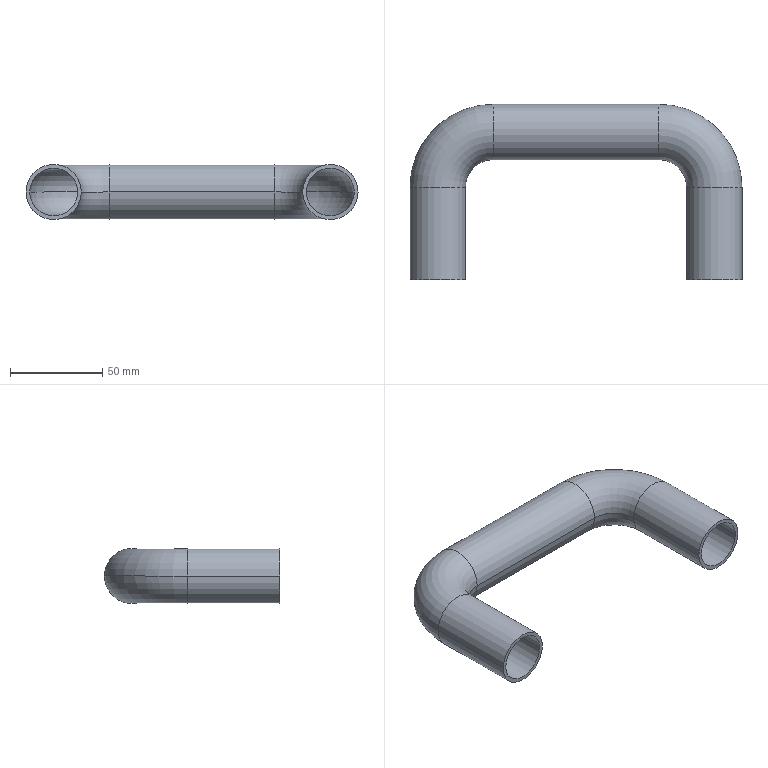Component | SolidWorks | CoverPlate-100_CoverHandle-1 | 1 solid | 22 faces | box 180 x 95 x 30 mm | volume 50007 mm3 | cylinder 12 | torus 8 | plane 2 | commonest cylinder face diameters 26 x6 30 x6 | material Plain Carbon Steel
build123d program:
from build123d import *

# Parameters (mm, degrees)
SWEEP_THIN1_PROFILE_R   = 15
SWEEP_THIN1_PROFILE_R_2 = 13


with BuildPart() as part:
    # Sweep-Thin1: sweep along a path in Sketch1
    with BuildLine(Plane(origin=(0, 0, 0), x_dir=(1, 0, 0), z_dir=(0, 1, 0))) as sweep_thin1_path:
        Line((0, 0), (0, 50))
        ThreePointArc((0, 50), (8.787, 71.213), (30, 80))
        Line((30, 80), (120, 80))
        ThreePointArc((120, 80), (141.213, 71.213), (150, 50))
        Line((150, 50), (150, 0))
    # Sweep-Thin1 profile (on start of the path) → Sweep-Thin1 (sweep)
    with BuildSketch(Plane(origin=(0, 0, 0), x_dir=(-1, 0, 0), z_dir=(0, 0, -1))):
        Circle(SWEEP_THIN1_PROFILE_R)
        Circle(SWEEP_THIN1_PROFILE_R_2, mode=Mode.SUBTRACT)
    sweep(path=sweep_thin1_path.line)


solid = part.part

# Placed as in the assembly
solid = solid.moved(Location((-455.465, 3543.733, 6089.043), (90, 0, 0)))
STEP:
#1=COLOUR_RGB('',0.7922,0.8196,0.9333);
#2=FILL_AREA_STYLE_COLOUR('',#1);
#3=FILL_AREA_STYLE('',(#2));
#4=SURFACE_STYLE_FILL_AREA(#3);
#5=SURFACE_SIDE_STYLE('',(#4));
#6=SURFACE_STYLE_USAGE(.BOTH.,#5);
#7=PRESENTATION_STYLE_ASSIGNMENT((#6));
#8=CARTESIAN_POINT('',(-13.207,142.155,239.726));
#9=VERTEX_POINT('',#8);
#10=CARTESIAN_POINT('',(-13.207,143.178,239.726));
#11=VERTEX_POINT('',#10);
#12=CARTESIAN_POINT('',(-13.207,142.667,239.726));
#13=DIRECTION('',(-1.,0.,0.));
#14=DIRECTION('',(0.,1.,0.));
#15=AXIS2_PLACEMENT_3D('',#12,#13,#14);
#16=CIRCLE('',#15,0.5118);
#17=EDGE_CURVE('',#9,#11,#16,.T.);
#18=ORIENTED_EDGE('',*,*,#17,.T.);
#19=CARTESIAN_POINT('',(-11.514,141.486,239.726));
#20=VERTEX_POINT('',#19);
#21=CARTESIAN_POINT('',(-13.207,141.486,239.726));
#22=DIRECTION('',(0.,0.,-1.));
#23=DIRECTION('',(0.,1.,0.));
#24=AXIS2_PLACEMENT_3D('',#21,#22,#23);
#25=CIRCLE('',#24,1.693);
#26=EDGE_CURVE('',#11,#20,#25,.T.);
#27=ORIENTED_EDGE('',*,*,#26,.T.);
#28=CARTESIAN_POINT('',(-12.538,141.486,239.726));
#29=VERTEX_POINT('',#28);
#30=CARTESIAN_POINT('',(-12.026,141.486,239.726));
#31=DIRECTION('',(-0.,1.,0.));
#32=DIRECTION('',(-1.,-0.,0.));
#33=AXIS2_PLACEMENT_3D('',#30,#31,#32);
#34=CIRCLE('',#33,0.5118);
#35=EDGE_CURVE('',#29,#20,#34,.T.);
#36=ORIENTED_EDGE('',*,*,#35,.F.);
#37=CARTESIAN_POINT('',(-13.207,141.486,239.726));
#38=DIRECTION('',(0.,0.,-1.));
#39=DIRECTION('',(0.,1.,0.));
#40=AXIS2_PLACEMENT_3D('',#37,#38,#39);
#41=CIRCLE('',#40,0.6693);
#42=EDGE_CURVE('',#9,#29,#41,.T.);
#43=ORIENTED_EDGE('',*,*,#42,.F.);
#44=EDGE_LOOP('',(#18,#27,#36,#43));
#45=FACE_OUTER_BOUND('',#44,.T.);
#46=CARTESIAN_POINT('',(-13.207,141.486,239.726));
#47=DIRECTION('',(0.,0.,-1.));
#48=DIRECTION('',(0.,1.,0.));
#49=AXIS2_PLACEMENT_3D('',#46,#47,#48);
#50=TOROIDAL_SURFACE('',#49,1.181,0.5118);
#51=ADVANCED_FACE('',(#45),#50,.F.);
#52=CARTESIAN_POINT('',(-17.42,141.486,239.726));
#53=VERTEX_POINT('',#52);
#54=CARTESIAN_POINT('',(-18.444,141.486,239.726));
#55=VERTEX_POINT('',#54);
#56=CARTESIAN_POINT('',(-17.932,141.486,239.726));
#57=DIRECTION('',(0.,-1.,-0.));
#58=DIRECTION('',(-1.,0.,0.));
#59=AXIS2_PLACEMENT_3D('',#56,#57,#58);
#60=CIRCLE('',#59,0.5118);
#61=EDGE_CURVE('',#53,#55,#60,.T.);
#62=ORIENTED_EDGE('',*,*,#61,.T.);
#63=CARTESIAN_POINT('',(-16.751,143.178,239.726));
#64=VERTEX_POINT('',#63);
#65=CARTESIAN_POINT('',(-16.751,141.486,239.726));
#66=DIRECTION('',(0.,0.,-1.));
#67=DIRECTION('',(0.,1.,0.));
#68=AXIS2_PLACEMENT_3D('',#65,#66,#67);
#69=CIRCLE('',#68,1.693);
#70=EDGE_CURVE('',#55,#64,#69,.T.);
#71=ORIENTED_EDGE('',*,*,#70,.T.);
#72=CARTESIAN_POINT('',(-16.751,142.155,239.726));
#73=VERTEX_POINT('',#72);
#74=CARTESIAN_POINT('',(-16.751,142.667,239.726));
#75=DIRECTION('',(-1.,0.,0.));
#76=DIRECTION('',(0.,-1.,0.));
#77=AXIS2_PLACEMENT_3D('',#74,#75,#76);
#78=CIRCLE('',#77,0.5118);
#79=EDGE_CURVE('',#73,#64,#78,.T.);
#80=ORIENTED_EDGE('',*,*,#79,.F.);
#81=CARTESIAN_POINT('',(-16.751,141.486,239.726));
#82=DIRECTION('',(0.,0.,-1.));
#83=DIRECTION('',(0.,1.,0.));
#84=AXIS2_PLACEMENT_3D('',#81,#82,#83);
#85=CIRCLE('',#84,0.6693);
#86=EDGE_CURVE('',#53,#73,#85,.T.);
#87=ORIENTED_EDGE('',*,*,#86,.F.);
#88=EDGE_LOOP('',(#62,#71,#80,#87));
#89=FACE_OUTER_BOUND('',#88,.T.);
#90=CARTESIAN_POINT('',(-16.751,141.486,239.726));
#91=DIRECTION('',(0.,0.,-1.));
#92=DIRECTION('',(0.,1.,0.));
#93=AXIS2_PLACEMENT_3D('',#90,#91,#92);
#94=TOROIDAL_SURFACE('',#93,1.181,0.5118);
#95=ADVANCED_FACE('',(#89),#94,.F.);
#96=CARTESIAN_POINT('',(-13.207,143.257,239.726));
#97=VERTEX_POINT('',#96);
#98=CARTESIAN_POINT('',(-13.207,142.076,239.726));
#99=VERTEX_POINT('',#98);
#100=CARTESIAN_POINT('',(-13.207,142.667,239.726));
#101=DIRECTION('',(-1.,0.,0.));
#102=DIRECTION('',(0.,-1.,0.));
#103=AXIS2_PLACEMENT_3D('',#100,#101,#102);
#104=CIRCLE('',#103,0.5906);
#105=EDGE_CURVE('',#97,#99,#104,.T.);
#106=ORIENTED_EDGE('',*,*,#105,.F.);
#107=CARTESIAN_POINT('',(-11.436,141.486,239.726));
#108=VERTEX_POINT('',#107);
#109=CARTESIAN_POINT('',(-13.207,141.486,239.726));
#110=DIRECTION('',(0.,0.,-1.));
#111=DIRECTION('',(0.,1.,0.));
#112=AXIS2_PLACEMENT_3D('',#109,#110,#111);
#113=CIRCLE('',#112,1.772);
#114=EDGE_CURVE('',#97,#108,#113,.T.);
#115=ORIENTED_EDGE('',*,*,#114,.T.);
#116=CARTESIAN_POINT('',(-12.617,141.486,239.726));
#117=VERTEX_POINT('',#116);
#118=CARTESIAN_POINT('',(-12.026,141.486,239.726));
#119=DIRECTION('',(0.,1.,0.));
#120=DIRECTION('',(-1.,0.,0.));
#121=AXIS2_PLACEMENT_3D('',#118,#119,#120);
#122=CIRCLE('',#121,0.5906);
#123=EDGE_CURVE('',#108,#117,#122,.T.);
#124=ORIENTED_EDGE('',*,*,#123,.T.);
#125=CARTESIAN_POINT('',(-13.207,141.486,239.726));
#126=DIRECTION('',(0.,0.,-1.));
#127=DIRECTION('',(0.,1.,0.));
#128=AXIS2_PLACEMENT_3D('',#125,#126,#127);
#129=CIRCLE('',#128,0.5906);
#130=EDGE_CURVE('',#99,#117,#129,.T.);
#131=ORIENTED_EDGE('',*,*,#130,.F.);
#132=EDGE_LOOP('',(#106,#115,#124,#131));
#133=FACE_OUTER_BOUND('',#132,.T.);
#134=CARTESIAN_POINT('',(-13.207,141.486,239.726));
#135=DIRECTION('',(0.,0.,-1.));
#136=DIRECTION('',(0.,1.,0.));
#137=AXIS2_PLACEMENT_3D('',#134,#135,#136);
#138=TOROIDAL_SURFACE('',#137,1.181,0.5906);
#139=ADVANCED_FACE('',(#133),#138,.T.);
#140=CARTESIAN_POINT('',(-18.522,141.486,239.726));
#141=VERTEX_POINT('',#140);
#142=CARTESIAN_POINT('',(-17.341,141.486,239.726));
#143=VERTEX_POINT('',#142);
#144=CARTESIAN_POINT('',(-17.932,141.486,239.726));
#145=DIRECTION('',(0.,-1.,-0.));
#146=DIRECTION('',(1.,0.,0.));
#147=AXIS2_PLACEMENT_3D('',#144,#145,#146);
#148=CIRCLE('',#147,0.5906);
#149=EDGE_CURVE('',#141,#143,#148,.T.);
#150=ORIENTED_EDGE('',*,*,#149,.F.);
#151=CARTESIAN_POINT('',(-16.751,143.257,239.726));
#152=VERTEX_POINT('',#151);
#153=CARTESIAN_POINT('',(-16.751,141.486,239.726));
#154=DIRECTION('',(0.,0.,-1.));
#155=DIRECTION('',(0.,1.,0.));
#156=AXIS2_PLACEMENT_3D('',#153,#154,#155);
#157=CIRCLE('',#156,1.772);
#158=EDGE_CURVE('',#141,#152,#157,.T.);
#159=ORIENTED_EDGE('',*,*,#158,.T.);
#160=CARTESIAN_POINT('',(-16.751,142.076,239.726));
#161=VERTEX_POINT('',#160);
#162=CARTESIAN_POINT('',(-16.751,142.667,239.726));
#163=DIRECTION('',(-1.,0.,0.));
#164=DIRECTION('',(0.,-1.,0.));
#165=AXIS2_PLACEMENT_3D('',#162,#163,#164);
#166=CIRCLE('',#165,0.5906);
#167=EDGE_CURVE('',#152,#161,#166,.T.);
#168=ORIENTED_EDGE('',*,*,#167,.T.);
#169=CARTESIAN_POINT('',(-16.751,141.486,239.726));
#170=DIRECTION('',(0.,0.,-1.));
#171=DIRECTION('',(0.,1.,0.));
#172=AXIS2_PLACEMENT_3D('',#169,#170,#171);
#173=CIRCLE('',#172,0.5906);
#174=EDGE_CURVE('',#143,#161,#173,.T.);
#175=ORIENTED_EDGE('',*,*,#174,.F.);
#176=EDGE_LOOP('',(#150,#159,#168,#175));
#177=FACE_OUTER_BOUND('',#176,.T.);
#178=CARTESIAN_POINT('',(-16.751,141.486,239.726));
#179=DIRECTION('',(0.,0.,-1.));
#180=DIRECTION('',(0.,1.,0.));
#181=AXIS2_PLACEMENT_3D('',#178,#179,#180);
#182=TOROIDAL_SURFACE('',#181,1.181,0.5906);
#183=ADVANCED_FACE('',(#177),#182,.T.);
#184=CARTESIAN_POINT('',(-12.026,141.486,239.726));
#185=DIRECTION('',(-0.,1.,0.));
#186=DIRECTION('',(-1.,-0.,0.));
#187=AXIS2_PLACEMENT_3D('',#184,#185,#186);
#188=CIRCLE('',#187,0.5118);
#189=EDGE_CURVE('',#20,#29,#188,.T.);
#190=ORIENTED_EDGE('',*,*,#189,.T.);
#191=CARTESIAN_POINT('',(-12.538,139.517,239.726));
#192=VERTEX_POINT('',#191);
#193=CARTESIAN_POINT('',(-12.538,141.486,239.726));
#194=DIRECTION('',(0.,-1.,-0.));
#195=VECTOR('',#194,39.37);
#196=LINE('',#193,#195);
#197=EDGE_CURVE('',#29,#192,#196,.T.);
#198=ORIENTED_EDGE('',*,*,#197,.T.);
#199=CARTESIAN_POINT('',(-11.514,139.517,239.726));
#200=VERTEX_POINT('',#199);
#201=CARTESIAN_POINT('',(-12.026,139.517,239.726));
#202=DIRECTION('',(0.,1.,0.));
#203=DIRECTION('',(-1.,0.,0.));
#204=AXIS2_PLACEMENT_3D('',#201,#202,#203);
#205=CIRCLE('',#204,0.5118);
#206=EDGE_CURVE('',#200,#192,#205,.T.);
#207=ORIENTED_EDGE('',*,*,#206,.F.);
#208=CARTESIAN_POINT('',(-11.514,141.486,239.726));
#209=DIRECTION('',(0.,-1.,-0.));
#210=VECTOR('',#209,39.37);
#211=LINE('',#208,#210);
#212=EDGE_CURVE('',#20,#200,#211,.T.);
#213=ORIENTED_EDGE('',*,*,#212,.F.);
#214=EDGE_LOOP('',(#190,#198,#207,#213));
#215=FACE_OUTER_BOUND('',#214,.T.);
#216=CARTESIAN_POINT('',(-12.026,141.486,239.726));
#217=DIRECTION('',(0.,-1.,-0.));
#218=DIRECTION('',(1.,0.,0.));
#219=AXIS2_PLACEMENT_3D('',#216,#217,#218);
#220=CYLINDRICAL_SURFACE('',#219,0.5118);
#221=ADVANCED_FACE('',(#215),#220,.F.);
#222=CARTESIAN_POINT('',(-16.751,142.667,239.726));
#223=DIRECTION('',(-1.,0.,0.));
#224=DIRECTION('',(0.,-1.,0.));
#225=AXIS2_PLACEMENT_3D('',#222,#223,#224);
#226=CIRCLE('',#225,0.5118);
#227=EDGE_CURVE('',#64,#73,#226,.T.);
#228=ORIENTED_EDGE('',*,*,#227,.T.);
#229=CARTESIAN_POINT('',(-16.751,142.155,239.726));
#230=DIRECTION('',(1.,0.,0.));
#231=VECTOR('',#230,39.37);
#232=LINE('',#229,#231);
#233=EDGE_CURVE('',#73,#9,#232,.T.);
#234=ORIENTED_EDGE('',*,*,#233,.T.);
#235=CARTESIAN_POINT('',(-13.207,142.667,239.726));
#236=DIRECTION('',(-1.,0.,0.));
#237=DIRECTION('',(0.,1.,0.));
#238=AXIS2_PLACEMENT_3D('',#235,#236,#237);
#239=CIRCLE('',#238,0.5118);
#240=EDGE_CURVE('',#11,#9,#239,.T.);
#241=ORIENTED_EDGE('',*,*,#240,.F.);
#242=CARTESIAN_POINT('',(-16.751,143.178,239.726));
#243=DIRECTION('',(1.,0.,0.));
#244=VECTOR('',#243,39.37);
#245=LINE('',#242,#244);
#246=EDGE_CURVE('',#64,#11,#245,.T.);
#247=ORIENTED_EDGE('',*,*,#246,.F.);
#248=EDGE_LOOP('',(#228,#234,#241,#247));
#249=FACE_OUTER_BOUND('',#248,.T.);
#250=CARTESIAN_POINT('',(-16.751,142.667,239.726));
#251=DIRECTION('',(1.,0.,0.));
#252=DIRECTION('',(0.,1.,0.));
#253=AXIS2_PLACEMENT_3D('',#250,#251,#252);
#254=CYLINDRICAL_SURFACE('',#253,0.5118);
#255=ADVANCED_FACE('',(#249),#254,.F.);
#256=CARTESIAN_POINT('',(-18.444,139.517,239.726));
#257=VERTEX_POINT('',#256);
#258=CARTESIAN_POINT('',(-17.42,139.517,239.726));
#259=VERTEX_POINT('',#258);
#260=CARTESIAN_POINT('',(-17.932,139.517,239.726));
#261=DIRECTION('',(0.,-1.,-0.));
#262=DIRECTION('',(1.,0.,0.));
#263=AXIS2_PLACEMENT_3D('',#260,#261,#262);
#264=CIRCLE('',#263,0.5118);
#265=EDGE_CURVE('',#257,#259,#264,.T.);
#266=ORIENTED_EDGE('',*,*,#265,.T.);
#267=CARTESIAN_POINT('',(-17.42,139.517,239.726));
#268=DIRECTION('',(0.,1.,0.));
#269=VECTOR('',#268,39.37);
#270=LINE('',#267,#269);
#271=EDGE_CURVE('',#259,#53,#270,.T.);
#272=ORIENTED_EDGE('',*,*,#271,.T.);
#273=CARTESIAN_POINT('',(-17.932,141.486,239.726));
#274=DIRECTION('',(0.,-1.,-0.));
#275=DIRECTION('',(-1.,0.,0.));
#276=AXIS2_PLACEMENT_3D('',#273,#274,#275);
#277=CIRCLE('',#276,0.5118);
#278=EDGE_CURVE('',#55,#53,#277,.T.);
#279=ORIENTED_EDGE('',*,*,#278,.F.);
#280=CARTESIAN_POINT('',(-18.444,139.517,239.726));
#281=DIRECTION('',(0.,1.,0.));
#282=VECTOR('',#281,39.37);
#283=LINE('',#280,#282);
#284=EDGE_CURVE('',#257,#55,#283,.T.);
#285=ORIENTED_EDGE('',*,*,#284,.F.);
#286=EDGE_LOOP('',(#266,#272,#279,#285));
#287=FACE_OUTER_BOUND('',#286,.T.);
#288=CARTESIAN_POINT('',(-17.932,139.517,239.726));
#289=DIRECTION('',(0.,1.,0.));
#290=DIRECTION('',(-1.,0.,0.));
#291=AXIS2_PLACEMENT_3D('',#288,#289,#290);
#292=CYLINDRICAL_SURFACE('',#291,0.5118);
#293=ADVANCED_FACE('',(#287),#292,.F.);
#294=CARTESIAN_POINT('',(-12.026,141.486,239.726));
#295=DIRECTION('',(0.,1.,0.));
#296=DIRECTION('',(-1.,0.,0.));
#297=AXIS2_PLACEMENT_3D('',#294,#295,#296);
#298=CIRCLE('',#297,0.5906);
#299=EDGE_CURVE('',#117,#108,#298,.T.);
#300=ORIENTED_EDGE('',*,*,#299,.F.);
#301=CARTESIAN_POINT('',(-12.617,139.517,239.726));
#302=VERTEX_POINT('',#301);
#303=CARTESIAN_POINT('',(-12.617,141.486,239.726));
#304=DIRECTION('',(0.,-1.,-0.));
#305=VECTOR('',#304,39.37);
#306=LINE('',#303,#305);
#307=EDGE_CURVE('',#117,#302,#306,.T.);
#308=ORIENTED_EDGE('',*,*,#307,.T.);
#309=CARTESIAN_POINT('',(-11.436,139.517,239.726));
#310=VERTEX_POINT('',#309);
#311=CARTESIAN_POINT('',(-12.026,139.517,239.726));
#312=DIRECTION('',(0.,1.,0.));
#313=DIRECTION('',(-1.,0.,0.));
#314=AXIS2_PLACEMENT_3D('',#311,#312,#313);
#315=CIRCLE('',#314,0.5906);
#316=EDGE_CURVE('',#302,#310,#315,.T.);
#317=ORIENTED_EDGE('',*,*,#316,.T.);
#318=CARTESIAN_POINT('',(-11.436,141.486,239.726));
#319=DIRECTION('',(0.,-1.,-0.));
#320=VECTOR('',#319,39.37);
#321=LINE('',#318,#320);
#322=EDGE_CURVE('',#108,#310,#321,.T.);
#323=ORIENTED_EDGE('',*,*,#322,.F.);
#324=EDGE_LOOP('',(#300,#308,#317,#323));
#325=FACE_OUTER_BOUND('',#324,.T.);
#326=CARTESIAN_POINT('',(-12.026,141.486,239.726));
#327=DIRECTION('',(0.,-1.,-0.));
#328=DIRECTION('',(1.,0.,0.));
#329=AXIS2_PLACEMENT_3D('',#326,#327,#328);
#330=CYLINDRICAL_SURFACE('',#329,0.5906);
#331=ADVANCED_FACE('',(#325),#330,.T.);
#332=CARTESIAN_POINT('',(-16.751,142.667,239.726));
#333=DIRECTION('',(-1.,0.,0.));
#334=DIRECTION('',(0.,-1.,0.));
#335=AXIS2_PLACEMENT_3D('',#332,#333,#334);
#336=CIRCLE('',#335,0.5906);
#337=EDGE_CURVE('',#161,#152,#336,.T.);
#338=ORIENTED_EDGE('',*,*,#337,.F.);
#339=CARTESIAN_POINT('',(-16.751,142.076,239.726));
#340=DIRECTION('',(1.,0.,0.));
#341=VECTOR('',#340,39.37);
#342=LINE('',#339,#341);
#343=EDGE_CURVE('',#161,#99,#342,.T.);
#344=ORIENTED_EDGE('',*,*,#343,.T.);
#345=CARTESIAN_POINT('',(-13.207,142.667,239.726));
#346=DIRECTION('',(-1.,0.,0.));
#347=DIRECTION('',(0.,-1.,0.));
#348=AXIS2_PLACEMENT_3D('',#345,#346,#347);
#349=CIRCLE('',#348,0.5906);
#350=EDGE_CURVE('',#99,#97,#349,.T.);
#351=ORIENTED_EDGE('',*,*,#350,.T.);
#352=CARTESIAN_POINT('',(-16.751,143.257,239.726));
#353=DIRECTION('',(1.,0.,0.));
#354=VECTOR('',#353,39.37);
#355=LINE('',#352,#354);
#356=EDGE_CURVE('',#152,#97,#355,.T.);
#357=ORIENTED_EDGE('',*,*,#356,.F.);
#358=EDGE_LOOP('',(#338,#344,#351,#357));
#359=FACE_OUTER_BOUND('',#358,.T.);
#360=CARTESIAN_POINT('',(-16.751,142.667,239.726));
#361=DIRECTION('',(1.,0.,0.));
#362=DIRECTION('',(0.,1.,0.));
#363=AXIS2_PLACEMENT_3D('',#360,#361,#362);
#364=CYLINDRICAL_SURFACE('',#363,0.5906);
#365=ADVANCED_FACE('',(#359),#364,.T.);
#366=CARTESIAN_POINT('',(-17.341,139.517,239.726));
#367=VERTEX_POINT('',#366);
#368=CARTESIAN_POINT('',(-18.522,139.517,239.726));
#369=VERTEX_POINT('',#368);
#370=CARTESIAN_POINT('',(-17.932,139.517,239.726));
#371=DIRECTION('',(0.,-1.,-0.));
#372=DIRECTION('',(1.,0.,0.));
#373=AXIS2_PLACEMENT_3D('',#370,#371,#372);
#374=CIRCLE('',#373,0.5906);
#375=EDGE_CURVE('',#367,#369,#374,.T.);
#376=ORIENTED_EDGE('',*,*,#375,.F.);
#377=CARTESIAN_POINT('',(-17.341,139.517,239.726));
#378=DIRECTION('',(0.,1.,0.));
#379=VECTOR('',#378,39.37);
#380=LINE('',#377,#379);
#381=EDGE_CURVE('',#367,#143,#380,.T.);
#382=ORIENTED_EDGE('',*,*,#381,.T.);
#383=CARTESIAN_POINT('',(-17.932,141.486,239.726));
#384=DIRECTION('',(0.,-1.,-0.));
#385=DIRECTION('',(1.,0.,0.));
#386=AXIS2_PLACEMENT_3D('',#383,#384,#385);
#387=CIRCLE('',#386,0.5906);
#388=EDGE_CURVE('',#143,#141,#387,.T.);
#389=ORIENTED_EDGE('',*,*,#388,.T.);
#390=CARTESIAN_POINT('',(-18.522,139.517,239.726));
#391=DIRECTION('',(0.,1.,0.));
#392=VECTOR('',#391,39.37);
#393=LINE('',#390,#392);
#394=EDGE_CURVE('',#369,#141,#393,.T.);
#395=ORIENTED_EDGE('',*,*,#394,.F.);
#396=EDGE_LOOP('',(#376,#382,#389,#395));
#397=FACE_OUTER_BOUND('',#396,.T.);
#398=CARTESIAN_POINT('',(-17.932,139.517,239.726));
#399=DIRECTION('',(0.,1.,0.));
#400=DIRECTION('',(-1.,0.,0.));
#401=AXIS2_PLACEMENT_3D('',#398,#399,#400);
#402=CYLINDRICAL_SURFACE('',#401,0.5906);
#403=ADVANCED_FACE('',(#397),#402,.T.);
#404=ORIENTED_EDGE('',*,*,#307,.F.);
#405=ORIENTED_EDGE('',*,*,#123,.F.);
#406=ORIENTED_EDGE('',*,*,#322,.T.);
#407=CARTESIAN_POINT('',(-12.026,139.517,239.726));
#408=DIRECTION('',(0.,1.,0.));
#409=DIRECTION('',(-1.,0.,0.));
#410=AXIS2_PLACEMENT_3D('',#407,#408,#409);
#411=CIRCLE('',#410,0.5906);
#412=EDGE_CURVE('',#310,#302,#411,.T.);
#413=ORIENTED_EDGE('',*,*,#412,.T.);
#414=EDGE_LOOP('',(#404,#405,#406,#413));
#415=FACE_OUTER_BOUND('',#414,.T.);
#416=CARTESIAN_POINT('',(-12.026,141.486,239.726));
#417=DIRECTION('',(0.,-1.,-0.));
#418=DIRECTION('',(1.,0.,0.));
#419=AXIS2_PLACEMENT_3D('',#416,#417,#418);
#420=CYLINDRICAL_SURFACE('',#419,0.5906);
#421=ADVANCED_FACE('',(#415),#420,.T.);
#422=ORIENTED_EDGE('',*,*,#114,.F.);
#423=ORIENTED_EDGE('',*,*,#350,.F.);
#424=ORIENTED_EDGE('',*,*,#130,.T.);
#425=ORIENTED_EDGE('',*,*,#299,.T.);
#426=EDGE_LOOP('',(#422,#423,#424,#425));
#427=FACE_OUTER_BOUND('',#426,.T.);
#428=CARTESIAN_POINT('',(-13.207,141.486,239.726));
#429=DIRECTION('',(0.,0.,-1.));
#430=DIRECTION('',(0.,1.,0.));
#431=AXIS2_PLACEMENT_3D('',#428,#429,#430);
#432=TOROIDAL_SURFACE('',#431,1.181,0.5906);
#433=ADVANCED_FACE('',(#427),#432,.T.);
#434=ORIENTED_EDGE('',*,*,#343,.F.);
#435=ORIENTED_EDGE('',*,*,#167,.F.);
#436=ORIENTED_EDGE('',*,*,#356,.T.);
#437=ORIENTED_EDGE('',*,*,#105,.T.);
#438=EDGE_LOOP('',(#434,#435,#436,#437));
#439=FACE_OUTER_BOUND('',#438,.T.);
#440=CARTESIAN_POINT('',(-16.751,142.667,239.726));
#441=DIRECTION('',(1.,0.,0.));
#442=DIRECTION('',(0.,1.,0.));
#443=AXIS2_PLACEMENT_3D('',#440,#441,#442);
#444=CYLINDRICAL_SURFACE('',#443,0.5906);
#445=ADVANCED_FACE('',(#439),#444,.T.);
#446=ORIENTED_EDGE('',*,*,#158,.F.);
#447=ORIENTED_EDGE('',*,*,#388,.F.);
#448=ORIENTED_EDGE('',*,*,#174,.T.);
#449=ORIENTED_EDGE('',*,*,#337,.T.);
#450=EDGE_LOOP('',(#446,#447,#448,#449));
#451=FACE_OUTER_BOUND('',#450,.T.);
#452=CARTESIAN_POINT('',(-16.751,141.486,239.726));
#453=DIRECTION('',(0.,0.,-1.));
#454=DIRECTION('',(0.,1.,0.));
#455=AXIS2_PLACEMENT_3D('',#452,#453,#454);
#456=TOROIDAL_SURFACE('',#455,1.181,0.5906);
#457=ADVANCED_FACE('',(#451),#456,.T.);
#458=ORIENTED_EDGE('',*,*,#381,.F.);
#459=CARTESIAN_POINT('',(-17.932,139.517,239.726));
#460=DIRECTION('',(0.,-1.,-0.));
#461=DIRECTION('',(1.,0.,0.));
#462=AXIS2_PLACEMENT_3D('',#459,#460,#461);
#463=CIRCLE('',#462,0.5906);
#464=EDGE_CURVE('',#369,#367,#463,.T.);
#465=ORIENTED_EDGE('',*,*,#464,.F.);
#466=ORIENTED_EDGE('',*,*,#394,.T.);
#467=ORIENTED_EDGE('',*,*,#149,.T.);
#468=EDGE_LOOP('',(#458,#465,#466,#467));
#469=FACE_OUTER_BOUND('',#468,.T.);
#470=CARTESIAN_POINT('',(-17.932,139.517,239.726));
#471=DIRECTION('',(0.,1.,0.));
#472=DIRECTION('',(-1.,0.,0.));
#473=AXIS2_PLACEMENT_3D('',#470,#471,#472);
#474=CYLINDRICAL_SURFACE('',#473,0.5906);
#475=ADVANCED_FACE('',(#469),#474,.T.);
#476=ORIENTED_EDGE('',*,*,#206,.T.);
#477=CARTESIAN_POINT('',(-12.026,139.517,239.726));
#478=DIRECTION('',(0.,1.,0.));
#479=DIRECTION('',(-1.,0.,0.));
#480=AXIS2_PLACEMENT_3D('',#477,#478,#479);
#481=CIRCLE('',#480,0.5118);
#482=EDGE_CURVE('',#192,#200,#481,.T.);
#483=ORIENTED_EDGE('',*,*,#482,.T.);
#484=EDGE_LOOP('',(#476,#483));
#485=FACE_BOUND('',#484,.T.);
#486=ORIENTED_EDGE('',*,*,#412,.F.);
#487=ORIENTED_EDGE('',*,*,#316,.F.);
#488=EDGE_LOOP('',(#486,#487));
#489=FACE_OUTER_BOUND('',#488,.T.);
#490=CARTESIAN_POINT('',(-12.026,139.517,239.726));
#491=DIRECTION('',(0.,1.,0.));
#492=DIRECTION('',(-1.,0.,0.));
#493=AXIS2_PLACEMENT_3D('',#490,#491,#492);
#494=PLANE('',#493);
#495=ADVANCED_FACE('',(#485,#489),#494,.F.);
#496=ORIENTED_EDGE('',*,*,#265,.F.);
#497=CARTESIAN_POINT('',(-17.932,139.517,239.726));
#498=DIRECTION('',(0.,-1.,-0.));
#499=DIRECTION('',(1.,0.,0.));
#500=AXIS2_PLACEMENT_3D('',#497,#498,#499);
#501=CIRCLE('',#500,0.5118);
#502=EDGE_CURVE('',#259,#257,#501,.T.);
#503=ORIENTED_EDGE('',*,*,#502,.F.);
#504=EDGE_LOOP('',(#496,#503));
#505=FACE_BOUND('',#504,.T.);
#506=ORIENTED_EDGE('',*,*,#464,.T.);
#507=ORIENTED_EDGE('',*,*,#375,.T.);
#508=EDGE_LOOP('',(#506,#507));
#509=FACE_OUTER_BOUND('',#508,.T.);
#510=CARTESIAN_POINT('',(-17.932,139.517,239.726));
#511=DIRECTION('',(0.,-1.,-0.));
#512=DIRECTION('',(1.,0.,0.));
#513=AXIS2_PLACEMENT_3D('',#510,#511,#512);
#514=PLANE('',#513);
#515=ADVANCED_FACE('',(#505,#509),#514,.T.);
#516=ORIENTED_EDGE('',*,*,#197,.F.);
#517=ORIENTED_EDGE('',*,*,#35,.T.);
#518=ORIENTED_EDGE('',*,*,#212,.T.);
#519=ORIENTED_EDGE('',*,*,#482,.F.);
#520=EDGE_LOOP('',(#516,#517,#518,#519));
#521=FACE_OUTER_BOUND('',#520,.T.);
#522=CARTESIAN_POINT('',(-12.026,141.486,239.726));
#523=DIRECTION('',(0.,-1.,-0.));
#524=DIRECTION('',(1.,0.,0.));
#525=AXIS2_PLACEMENT_3D('',#522,#523,#524);
#526=CYLINDRICAL_SURFACE('',#525,0.5118);
#527=ADVANCED_FACE('',(#521),#526,.F.);
#528=ORIENTED_EDGE('',*,*,#26,.F.);
#529=ORIENTED_EDGE('',*,*,#240,.T.);
#530=ORIENTED_EDGE('',*,*,#42,.T.);
#531=ORIENTED_EDGE('',*,*,#189,.F.);
#532=EDGE_LOOP('',(#528,#529,#530,#531));
#533=FACE_OUTER_BOUND('',#532,.T.);
#534=CARTESIAN_POINT('',(-13.207,141.486,239.726));
#535=DIRECTION('',(0.,0.,-1.));
#536=DIRECTION('',(0.,1.,0.));
#537=AXIS2_PLACEMENT_3D('',#534,#535,#536);
#538=TOROIDAL_SURFACE('',#537,1.181,0.5118);
#539=ADVANCED_FACE('',(#533),#538,.F.);
#540=ORIENTED_EDGE('',*,*,#233,.F.);
#541=ORIENTED_EDGE('',*,*,#79,.T.);
#542=ORIENTED_EDGE('',*,*,#246,.T.);
#543=ORIENTED_EDGE('',*,*,#17,.F.);
#544=EDGE_LOOP('',(#540,#541,#542,#543));
#545=FACE_OUTER_BOUND('',#544,.T.);
#546=CARTESIAN_POINT('',(-16.751,142.667,239.726));
#547=DIRECTION('',(1.,0.,0.));
#548=DIRECTION('',(0.,1.,0.));
#549=AXIS2_PLACEMENT_3D('',#546,#547,#548);
#550=CYLINDRICAL_SURFACE('',#549,0.5118);
#551=ADVANCED_FACE('',(#545),#550,.F.);
#552=ORIENTED_EDGE('',*,*,#70,.F.);
#553=ORIENTED_EDGE('',*,*,#278,.T.);
#554=ORIENTED_EDGE('',*,*,#86,.T.);
#555=ORIENTED_EDGE('',*,*,#227,.F.);
#556=EDGE_LOOP('',(#552,#553,#554,#555));
#557=FACE_OUTER_BOUND('',#556,.T.);
#558=CARTESIAN_POINT('',(-16.751,141.486,239.726));
#559=DIRECTION('',(0.,0.,-1.));
#560=DIRECTION('',(0.,1.,0.));
#561=AXIS2_PLACEMENT_3D('',#558,#559,#560);
#562=TOROIDAL_SURFACE('',#561,1.181,0.5118);
#563=ADVANCED_FACE('',(#557),#562,.F.);
#564=ORIENTED_EDGE('',*,*,#271,.F.);
#565=ORIENTED_EDGE('',*,*,#502,.T.);
#566=ORIENTED_EDGE('',*,*,#284,.T.);
#567=ORIENTED_EDGE('',*,*,#61,.F.);
#568=EDGE_LOOP('',(#564,#565,#566,#567));
#569=FACE_OUTER_BOUND('',#568,.T.);
#570=CARTESIAN_POINT('',(-17.932,139.517,239.726));
#571=DIRECTION('',(0.,1.,0.));
#572=DIRECTION('',(-1.,0.,0.));
#573=AXIS2_PLACEMENT_3D('',#570,#571,#572);
#574=CYLINDRICAL_SURFACE('',#573,0.5118);
#575=ADVANCED_FACE('',(#569),#574,.F.);
#576=CLOSED_SHELL('',(#51,#95,#139,#183,#221,#255,#293,#331,#365,#403,#421,#433,#445,#457,#475,#495,#515,#527,#539,#551,#563,#575));
#577=MANIFOLD_SOLID_BREP('',#576);
#578=STYLED_ITEM('',(#7),#577);
#579=PRESENTATION_LAYER_ASSIGNMENT('','',(#578));
#580=CARTESIAN_POINT('',(0.,0.,0.));
#581=DIRECTION('',(0.,0.,1.));
#582=DIRECTION('',(1.,0.,0.));
#583=AXIS2_PLACEMENT_3D('',#580,#581,#582);
#584=(LENGTH_UNIT()NAMED_UNIT(*)SI_UNIT($,.METRE.));
#585=LENGTH_MEASURE_WITH_UNIT(LENGTH_MEASURE(0.0254),#584);
#586=DIMENSIONAL_EXPONENTS(1.,0.,0.,0.,0.,0.,0.);
#587=(CONVERSION_BASED_UNIT('',#585)LENGTH_UNIT()NAMED_UNIT(#586));
#588=UNCERTAINTY_MEASURE_WITH_UNIT(LENGTH_MEASURE(0.00001),#587,'','');
#589=(NAMED_UNIT(*)PLANE_ANGLE_UNIT()SI_UNIT($,.RADIAN.));
#590=(NAMED_UNIT(*)SI_UNIT($,.STERADIAN.)SOLID_ANGLE_UNIT());
#591=(GEOMETRIC_REPRESENTATION_CONTEXT(3)GLOBAL_UNCERTAINTY_ASSIGNED_CONTEXT((#588))GLOBAL_UNIT_ASSIGNED_CONTEXT((#587,#589,#590))REPRESENTATION_CONTEXT('',''));
#592=ADVANCED_BREP_SHAPE_REPRESENTATION('',(#577,#583),#591);
#593=(LENGTH_UNIT()NAMED_UNIT(*)SI_UNIT($,.METRE.));
#594=LENGTH_MEASURE_WITH_UNIT(LENGTH_MEASURE(0.0254),#593);
#595=DIMENSIONAL_EXPONENTS(1.,0.,0.,0.,0.,0.,0.);
#596=(CONVERSION_BASED_UNIT('',#594)LENGTH_UNIT()NAMED_UNIT(#595));
#597=UNCERTAINTY_MEASURE_WITH_UNIT(LENGTH_MEASURE(0.00001),#596,'','');
#598=(NAMED_UNIT(*)PLANE_ANGLE_UNIT()SI_UNIT($,.RADIAN.));
#599=(NAMED_UNIT(*)SI_UNIT($,.STERADIAN.)SOLID_ANGLE_UNIT());
#600=(GEOMETRIC_REPRESENTATION_CONTEXT(3)GLOBAL_UNCERTAINTY_ASSIGNED_CONTEXT((#597))GLOBAL_UNIT_ASSIGNED_CONTEXT((#596,#598,#599))REPRESENTATION_CONTEXT('',''));
#601=MECHANICAL_DESIGN_GEOMETRIC_PRESENTATION_REPRESENTATION('',(#578),#600);